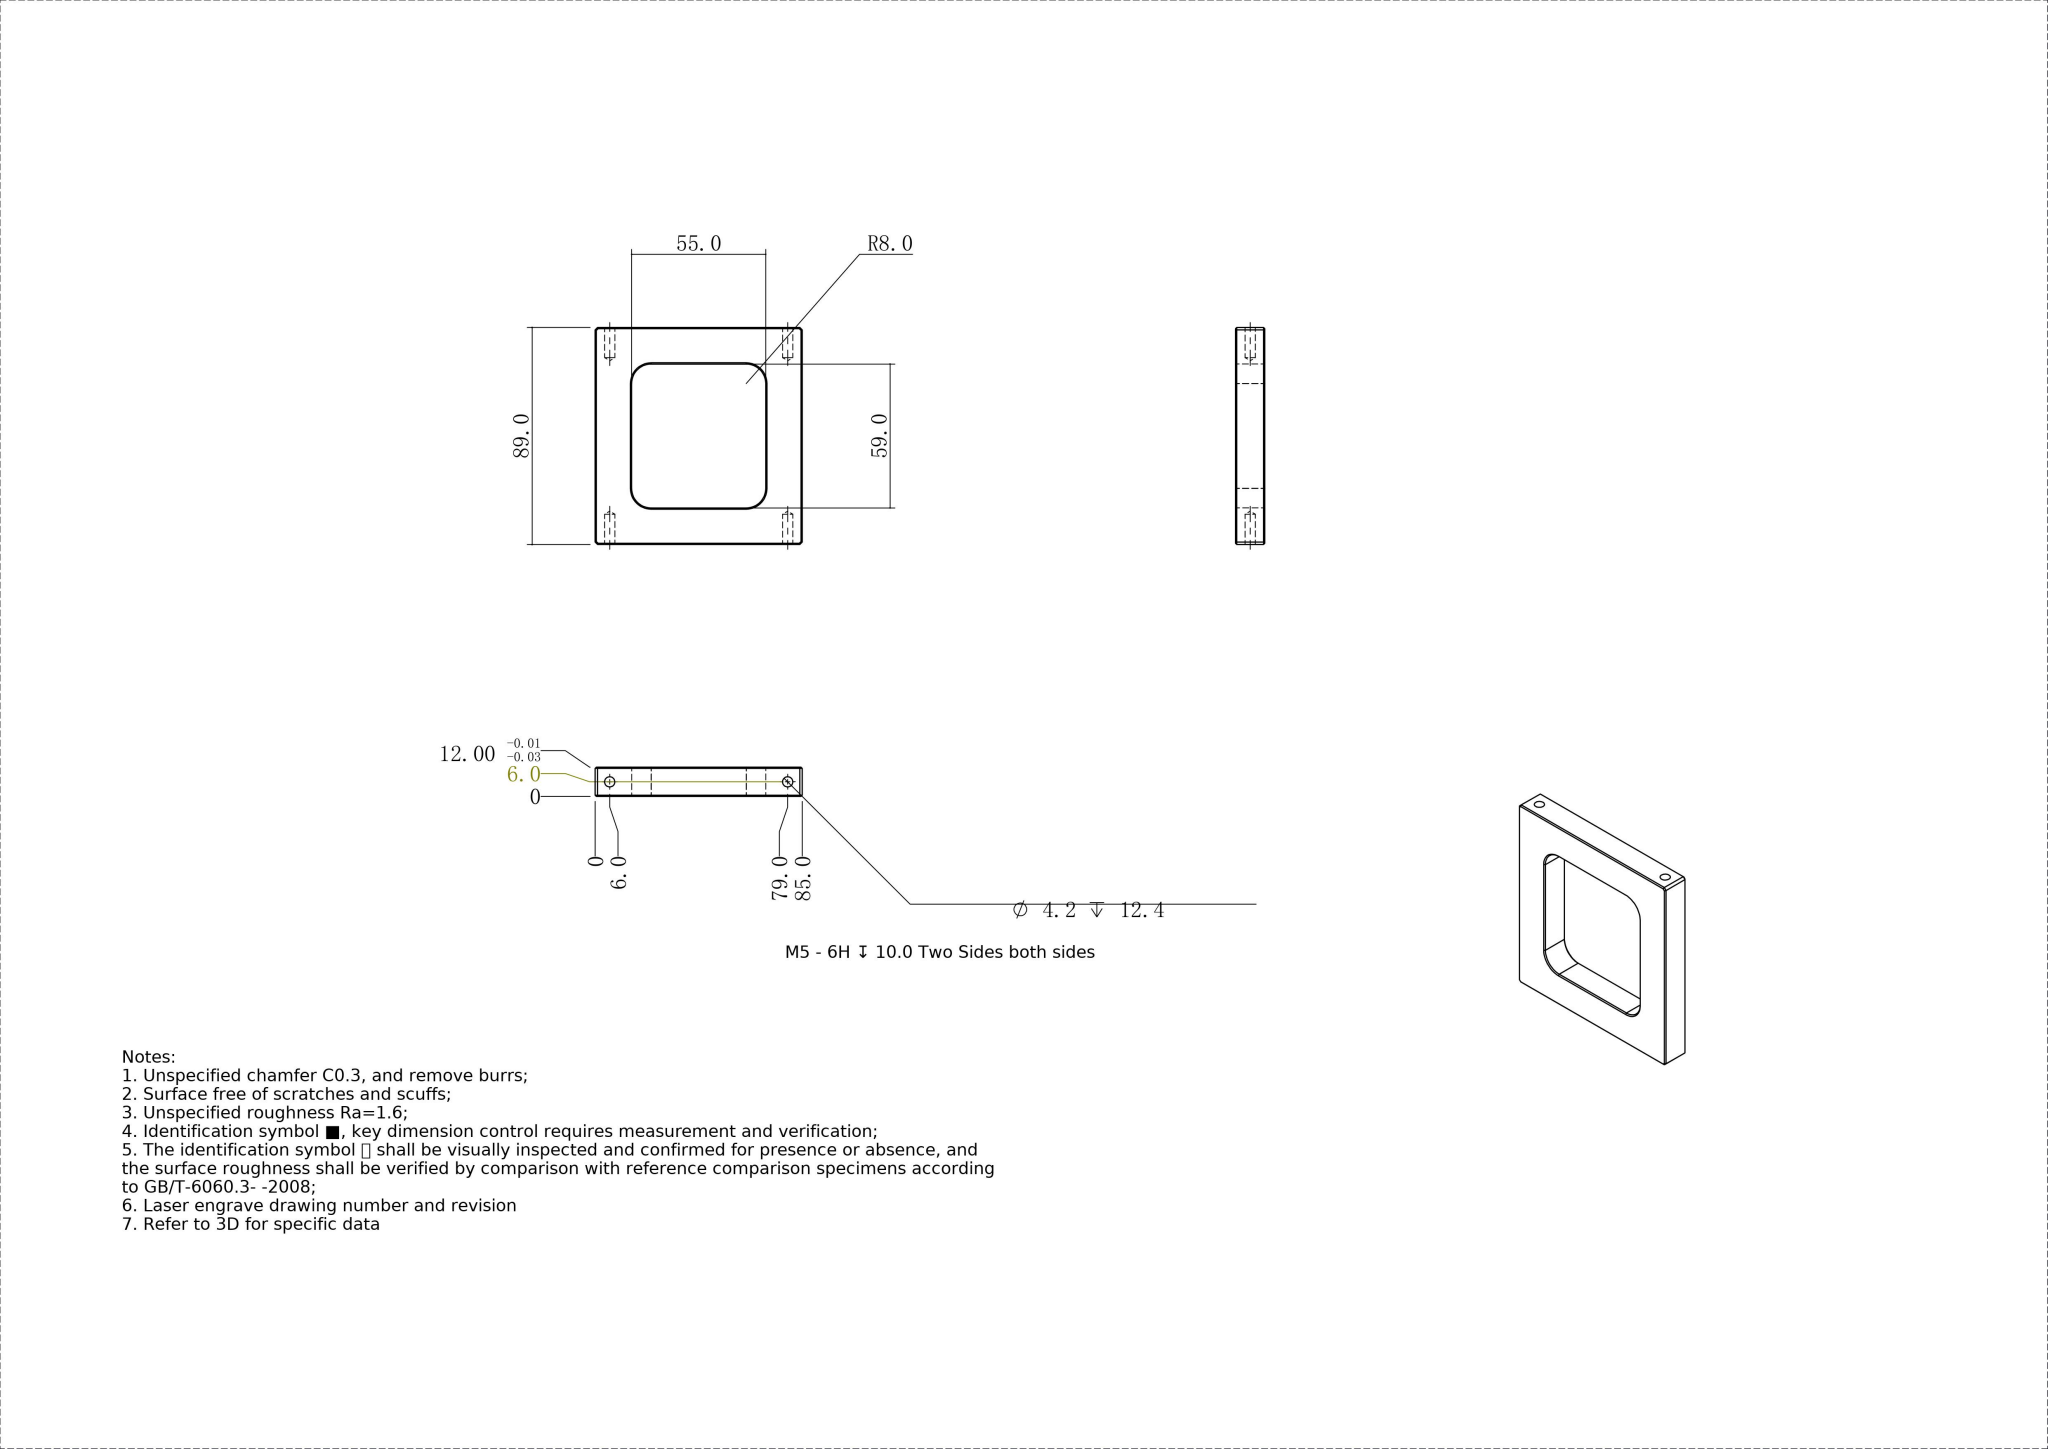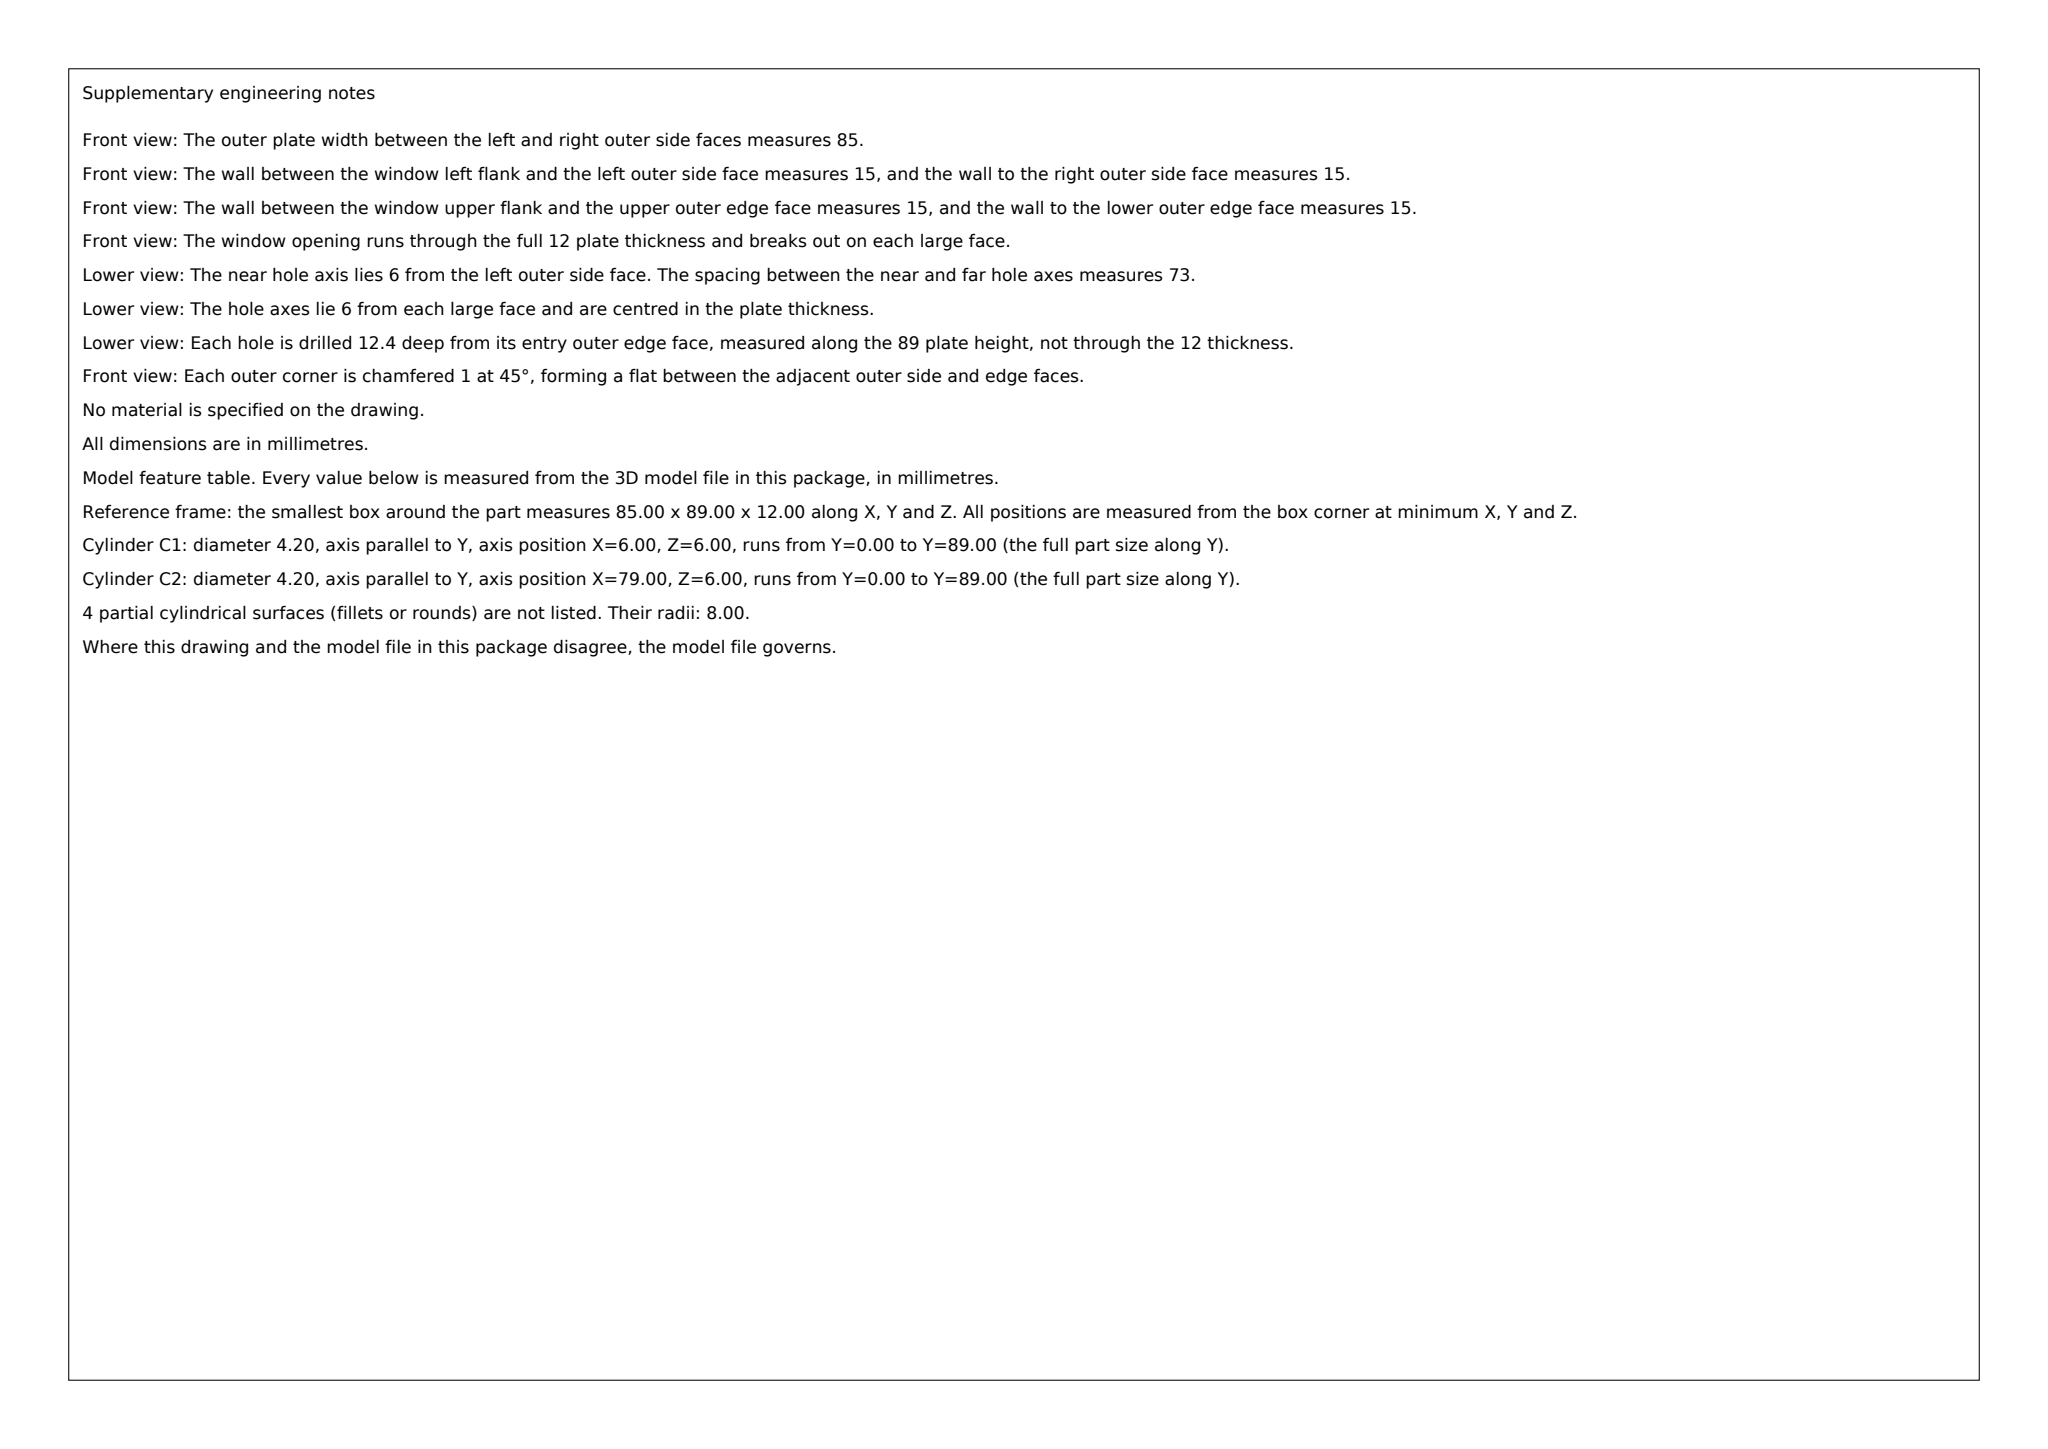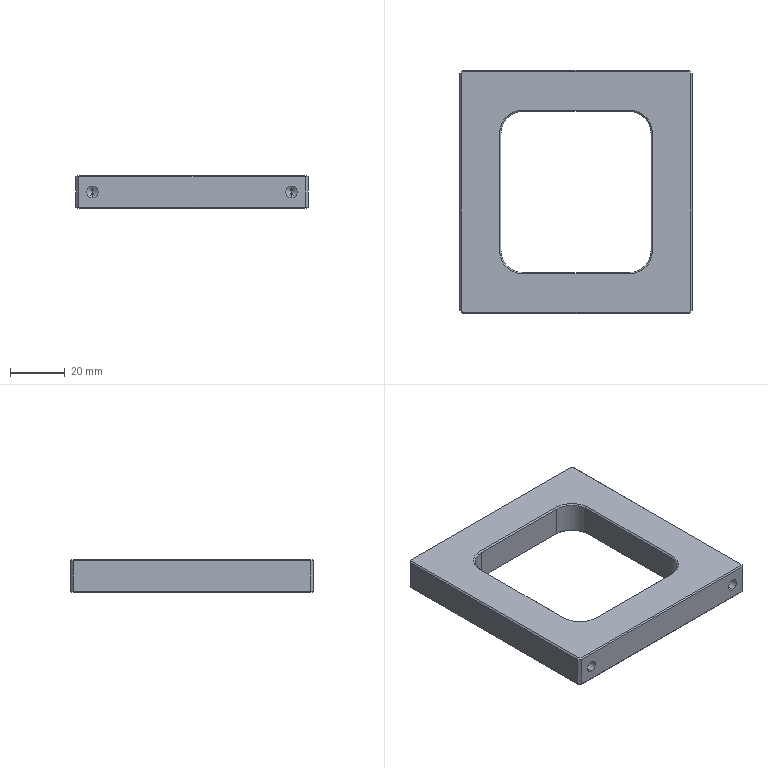Part | SolidWorks | mm | 1 solid | 66 faces | box 85 x 89 x 12 mm | volume 51625 mm3 | plane 38 | cone 16 | cylinder 12 | commonest cylinder face diameters 4.2 x8 16 x4
Drawing notes:
OVERALL 85.0 X 89.0 X 12.0 THK | from the solid: bbox_xyz [85.0, 89.0, 12.0]
POCKET 55.0 X 59.0 R8.0 DP 11.0 BLIND, FLOOR 1.0 | from the solid: R8 corner cyls dia16 axis Z len 11.0; walls x=15/70 (55), y=15/74 (59); bbox z=12.0
4X M5-6H DP 10.0, TAP DRILL Ø4.2 DP 12.4, X=6.0 & 79.0, Z=6.0 CL, TOP & BTM EDGES | from the solid: cyl dia4.2 axis Y at (x=6.0,z=6.0) & (x=79.0,z=6.0) len 12.4; 118° drill point cones ref dia 4.2
8X CSK Ø17.0 X 90° AT Ø4.2 ENTRIES, TOP & BTM EDGES | from the solid: cones[included_angle,ref_dia]=[90.0,17.0,8] at the Ø4.2 tap-drill entries, axis Y
build123d program:
from build123d import *

# Parameters (mm, degrees)
SKETCH1_W                  = 85
SKETCH1_H                  = 89
BOSS_EXTRUDE1_DEPTH        = 6
M5_TAPPED_HOLE1_AT_2_COUNT = 2
M5_TAPPED_HOLE1_AT_2_PITCH = 73
SKETCH4_W                  = 55
SKETCH4_H                  = 59
CUT_EXTRUDE1_DEPTH         = 36
FILLET1_R                  = 8
CHAMFER1_SIZE              = 1
CHAMFER2_SIZE              = 0.5


with BuildPart() as part:
    # Sketch1 → Boss-Extrude1 (new, symmetric)
    with BuildSketch(Plane.XY):
        Rectangle(SKETCH1_W, SKETCH1_H)
    extrude(amount=BOSS_EXTRUDE1_DEPTH, both=True)

    # Sketch3 → M5 Tapped Hole1 (revolve, cut)
    with BuildSketch(Plane(origin=(-36.5, 44.5, 0), x_dir=(0, 0, 1), z_dir=(1, 0, 0))):
        Polygon((0, 0), (0, 13.662), (2.1, 12.4), (2.1, 0), align=None)
    m5_tapped_hole1 = revolve(axis=Axis((-36.5, 50.85, 0), (0, -1, 0)), mode=Mode.SUBTRACT)

    # M5 Tapped Hole1 at 2: M5 Tapped Hole1 ×2
    with Locations(*[(i * M5_TAPPED_HOLE1_AT_2_PITCH, 0, 0) for i in range(1, M5_TAPPED_HOLE1_AT_2_COUNT)]):
        add(m5_tapped_hole1, mode=Mode.SUBTRACT)

    # Mirror1: M5 Tapped Hole1 across plane
    add(m5_tapped_hole1.mirror(Plane.ZX), mode=Mode.SUBTRACT)

    # Mirror1 copy 1 sketch → Mirror1 copy 1 (revolve, cut)
    with BuildSketch(Plane(origin=(36.5, -44.5, 0), x_dir=(0, 0, 1), z_dir=(1, 0, 0))):
        Polygon((0, 0), (0, -13.662), (2.1, -12.4), (2.1, 0), align=None)
    revolve(axis=Axis((36.5, -50.85, 0), (0, -1, 0)), mode=Mode.SUBTRACT)

    # Sketch4 → Cut-Extrude1 (cut)
    with BuildSketch(Plane(origin=(0, 0, -6), x_dir=(-1, 0, 0), z_dir=(0, 0, -1))):
        Rectangle(SKETCH4_W, SKETCH4_H)
    extrude(amount=-CUT_EXTRUDE1_DEPTH, mode=Mode.SUBTRACT)

    # Fillet1
    fillet1_edges = [part.edges().sort_by_distance(p)[0] for p in [
        (-27.5, 29.5, 0),
        (-27.5, -29.5, 0),
        (27.5, -29.5, 0),
        (27.5, 29.5, 0),
    ]]
    fillet(fillet1_edges, radius=FILLET1_R)

    # Chamfer1
    chamfer1_edges = [part.edges().sort_by_distance(p)[0] for p in [
        (42.5, -44.5, 0),
        (-42.5, -44.5, 0),
        (-42.5, 44.5, 0),
        (42.5, 44.5, 0),
    ]]
    chamfer(chamfer1_edges, length=CHAMFER1_SIZE)

    # Chamfer2
    chamfer2_edges = [part.edges().sort_by_distance(p)[0] for p in [
        (-42.5, 0, 6),
        (42.5, 0, -6),
        (0, -44.5, -6),
        (0, 44.5, -6),
        (42, -44, -6),
        (-42, -44, -6),
        (42, 44, -6),
        (-42, 44, -6),
        (0, 44.5, 6),
        (42.5, 0, 6),
        (0, -44.5, 6),
        (42, -44, 6),
        (-42, -44, 6),
        (42, 44, 6),
        (-42, 44, 6),
        (-27.5, 0, -6),
        (-27.5, 0, 6),
        (0, -29.5, -6),
        (0, -29.5, 6),
        (27.5, 0, -6),
        (27.5, 0, 6),
        (0, 29.5, -6),
        (0, 29.5, 6),
        (-25.157, -27.157, -6),
        (-25.157, -27.157, 6),
        (25.157, -27.157, -6),
        (25.157, -27.157, 6),
        (25.157, 27.157, -6),
        (25.157, 27.157, 6),
        (-25.157, 27.157, -6),
        (-25.157, 27.157, 6),
        (-42.5, 0, -6),
    ]]
    chamfer(chamfer2_edges, length=CHAMFER2_SIZE)


solid = part.part